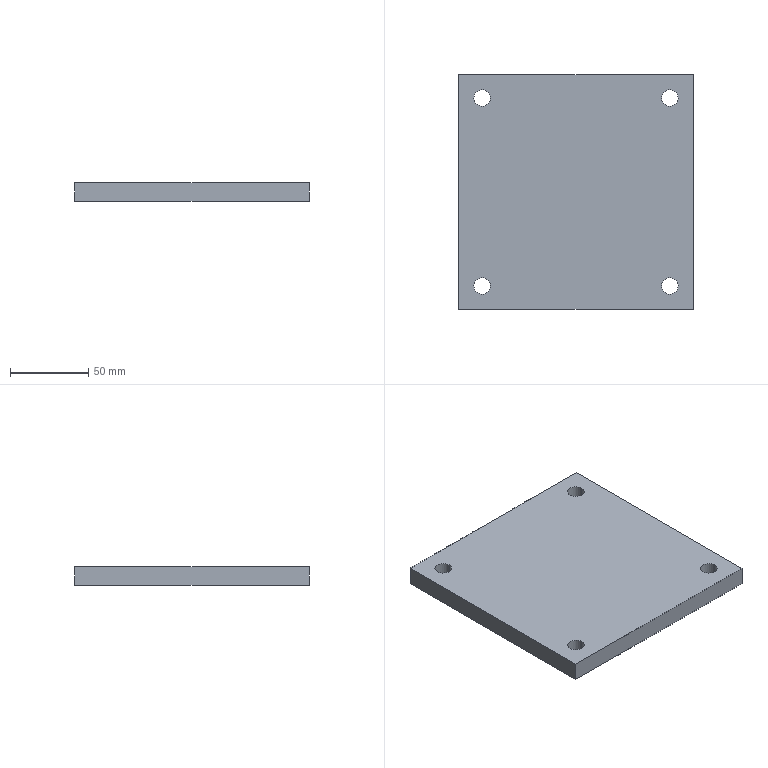Component | SolidWorks | CSFA2082 074-1 | 1 solid | 14 faces | box 150 x 150 x 12 mm | volume 265844 mm3 | cylinder 8 | plane 6 | commonest cylinder face diameters 10.5 x8
build123d program:
from build123d import *

# Parameters (mm, degrees)
SKETCH1_W                        = 150
SKETCH1_H                        = 150
EXTRUDE1_DEPTH                   = 12
F_10_5_10_5_DIAMETER_HOLE1_D     = 10.5
F_10_5_10_5_DIAMETER_HOLE1_DEPTH = 71
F_10_5_10_5_DIAMETER_HOLE1_TIP   = 3.155


with BuildPart() as part:
    # Sketch1 → Extrude1 (new body)
    with BuildSketch(Plane.XY):
        Rectangle(SKETCH1_W, SKETCH1_H)
    extrude(amount=EXTRUDE1_DEPTH)

    # 10.5 _10.5_ Diameter Hole1
    with Locations(Plane.XY.offset(12)):
        with Locations((-60, 60), (-60, -60), (60, -60), (60, 60)):
            Hole(F_10_5_10_5_DIAMETER_HOLE1_D / 2, depth=F_10_5_10_5_DIAMETER_HOLE1_DEPTH)
            with Locations((0, 0, -(F_10_5_10_5_DIAMETER_HOLE1_DEPTH + F_10_5_10_5_DIAMETER_HOLE1_TIP / 2))):  # 118° drill point
                Cone(0, F_10_5_10_5_DIAMETER_HOLE1_D / 2, F_10_5_10_5_DIAMETER_HOLE1_TIP, mode=Mode.SUBTRACT)


solid = part.part

# Placed as in the assembly
solid = solid.moved(Location((172.551, -218.176, 585), (0, 0, 0)))
STEP:
#1=COLOUR_RGB('',0.7922,0.8196,0.9333);
#2=FILL_AREA_STYLE_COLOUR('',#1);
#3=FILL_AREA_STYLE('',(#2));
#4=SURFACE_STYLE_FILL_AREA(#3);
#5=SURFACE_SIDE_STYLE('',(#4));
#6=SURFACE_STYLE_USAGE(.BOTH.,#5);
#7=PRESENTATION_STYLE_ASSIGNMENT((#6));
#8=CARTESIAN_POINT('',(4.638,-6.227,23.031));
#9=VERTEX_POINT('',#8);
#10=CARTESIAN_POINT('',(4.224,-6.227,23.031));
#11=VERTEX_POINT('',#10);
#12=CARTESIAN_POINT('',(4.431,-6.227,23.031));
#13=DIRECTION('',(0.,0.,-1.));
#14=DIRECTION('',(-1.,0.,0.));
#15=AXIS2_PLACEMENT_3D('',#12,#13,#14);
#16=CIRCLE('',#15,0.2067);
#17=EDGE_CURVE('',#9,#11,#16,.T.);
#18=ORIENTED_EDGE('',*,*,#17,.T.);
#19=CARTESIAN_POINT('',(4.224,-6.227,23.504));
#20=VERTEX_POINT('',#19);
#21=CARTESIAN_POINT('',(4.224,-6.227,23.504));
#22=DIRECTION('',(0.,0.,1.));
#23=VECTOR('',#22,39.37);
#24=LINE('',#21,#23);
#25=EDGE_CURVE('',#11,#20,#24,.T.);
#26=ORIENTED_EDGE('',*,*,#25,.T.);
#27=CARTESIAN_POINT('',(4.638,-6.227,23.504));
#28=VERTEX_POINT('',#27);
#29=CARTESIAN_POINT('',(4.431,-6.227,23.504));
#30=DIRECTION('',(0.,0.,1.));
#31=DIRECTION('',(1.,0.,0.));
#32=AXIS2_PLACEMENT_3D('',#29,#30,#31);
#33=CIRCLE('',#32,0.2067);
#34=EDGE_CURVE('',#20,#28,#33,.T.);
#35=ORIENTED_EDGE('',*,*,#34,.T.);
#36=CARTESIAN_POINT('',(4.638,-6.227,23.504));
#37=DIRECTION('',(0.,0.,1.));
#38=VECTOR('',#37,39.37);
#39=LINE('',#36,#38);
#40=EDGE_CURVE('',#9,#28,#39,.T.);
#41=ORIENTED_EDGE('',*,*,#40,.F.);
#42=EDGE_LOOP('',(#18,#26,#35,#41));
#43=FACE_OUTER_BOUND('',#42,.T.);
#44=CARTESIAN_POINT('',(4.431,-6.227,23.504));
#45=DIRECTION('',(0.,0.,1.));
#46=DIRECTION('',(1.,0.,0.));
#47=AXIS2_PLACEMENT_3D('',#44,#45,#46);
#48=CYLINDRICAL_SURFACE('',#47,0.2067);
#49=ADVANCED_FACE('',(#43),#48,.F.);
#50=CARTESIAN_POINT('',(4.638,-10.952,23.031));
#51=VERTEX_POINT('',#50);
#52=CARTESIAN_POINT('',(4.224,-10.952,23.031));
#53=VERTEX_POINT('',#52);
#54=CARTESIAN_POINT('',(4.431,-10.952,23.031));
#55=DIRECTION('',(0.,0.,-1.));
#56=DIRECTION('',(-1.,0.,0.));
#57=AXIS2_PLACEMENT_3D('',#54,#55,#56);
#58=CIRCLE('',#57,0.2067);
#59=EDGE_CURVE('',#51,#53,#58,.T.);
#60=ORIENTED_EDGE('',*,*,#59,.T.);
#61=CARTESIAN_POINT('',(4.224,-10.952,23.504));
#62=VERTEX_POINT('',#61);
#63=CARTESIAN_POINT('',(4.224,-10.952,23.504));
#64=DIRECTION('',(0.,0.,1.));
#65=VECTOR('',#64,39.37);
#66=LINE('',#63,#65);
#67=EDGE_CURVE('',#53,#62,#66,.T.);
#68=ORIENTED_EDGE('',*,*,#67,.T.);
#69=CARTESIAN_POINT('',(4.638,-10.952,23.504));
#70=VERTEX_POINT('',#69);
#71=CARTESIAN_POINT('',(4.431,-10.952,23.504));
#72=DIRECTION('',(0.,0.,1.));
#73=DIRECTION('',(1.,0.,0.));
#74=AXIS2_PLACEMENT_3D('',#71,#72,#73);
#75=CIRCLE('',#74,0.2067);
#76=EDGE_CURVE('',#62,#70,#75,.T.);
#77=ORIENTED_EDGE('',*,*,#76,.T.);
#78=CARTESIAN_POINT('',(4.638,-10.952,23.504));
#79=DIRECTION('',(0.,0.,1.));
#80=VECTOR('',#79,39.37);
#81=LINE('',#78,#80);
#82=EDGE_CURVE('',#51,#70,#81,.T.);
#83=ORIENTED_EDGE('',*,*,#82,.F.);
#84=EDGE_LOOP('',(#60,#68,#77,#83));
#85=FACE_OUTER_BOUND('',#84,.T.);
#86=CARTESIAN_POINT('',(4.431,-10.952,23.504));
#87=DIRECTION('',(0.,0.,1.));
#88=DIRECTION('',(1.,0.,0.));
#89=AXIS2_PLACEMENT_3D('',#86,#87,#88);
#90=CYLINDRICAL_SURFACE('',#89,0.2067);
#91=ADVANCED_FACE('',(#85),#90,.F.);
#92=CARTESIAN_POINT('',(9.362,-10.952,23.031));
#93=VERTEX_POINT('',#92);
#94=CARTESIAN_POINT('',(8.949,-10.952,23.031));
#95=VERTEX_POINT('',#94);
#96=CARTESIAN_POINT('',(9.156,-10.952,23.031));
#97=DIRECTION('',(0.,0.,-1.));
#98=DIRECTION('',(-1.,0.,0.));
#99=AXIS2_PLACEMENT_3D('',#96,#97,#98);
#100=CIRCLE('',#99,0.2067);
#101=EDGE_CURVE('',#93,#95,#100,.T.);
#102=ORIENTED_EDGE('',*,*,#101,.T.);
#103=CARTESIAN_POINT('',(8.949,-10.952,23.504));
#104=VERTEX_POINT('',#103);
#105=CARTESIAN_POINT('',(8.949,-10.952,23.504));
#106=DIRECTION('',(0.,0.,1.));
#107=VECTOR('',#106,39.37);
#108=LINE('',#105,#107);
#109=EDGE_CURVE('',#95,#104,#108,.T.);
#110=ORIENTED_EDGE('',*,*,#109,.T.);
#111=CARTESIAN_POINT('',(9.362,-10.952,23.504));
#112=VERTEX_POINT('',#111);
#113=CARTESIAN_POINT('',(9.156,-10.952,23.504));
#114=DIRECTION('',(0.,0.,1.));
#115=DIRECTION('',(1.,0.,0.));
#116=AXIS2_PLACEMENT_3D('',#113,#114,#115);
#117=CIRCLE('',#116,0.2067);
#118=EDGE_CURVE('',#104,#112,#117,.T.);
#119=ORIENTED_EDGE('',*,*,#118,.T.);
#120=CARTESIAN_POINT('',(9.362,-10.952,23.504));
#121=DIRECTION('',(0.,0.,1.));
#122=VECTOR('',#121,39.37);
#123=LINE('',#120,#122);
#124=EDGE_CURVE('',#93,#112,#123,.T.);
#125=ORIENTED_EDGE('',*,*,#124,.F.);
#126=EDGE_LOOP('',(#102,#110,#119,#125));
#127=FACE_OUTER_BOUND('',#126,.T.);
#128=CARTESIAN_POINT('',(9.156,-10.952,23.504));
#129=DIRECTION('',(0.,0.,1.));
#130=DIRECTION('',(1.,0.,0.));
#131=AXIS2_PLACEMENT_3D('',#128,#129,#130);
#132=CYLINDRICAL_SURFACE('',#131,0.2067);
#133=ADVANCED_FACE('',(#127),#132,.F.);
#134=CARTESIAN_POINT('',(9.362,-6.227,23.031));
#135=VERTEX_POINT('',#134);
#136=CARTESIAN_POINT('',(8.949,-6.227,23.031));
#137=VERTEX_POINT('',#136);
#138=CARTESIAN_POINT('',(9.156,-6.227,23.031));
#139=DIRECTION('',(0.,0.,-1.));
#140=DIRECTION('',(-1.,0.,0.));
#141=AXIS2_PLACEMENT_3D('',#138,#139,#140);
#142=CIRCLE('',#141,0.2067);
#143=EDGE_CURVE('',#135,#137,#142,.T.);
#144=ORIENTED_EDGE('',*,*,#143,.T.);
#145=CARTESIAN_POINT('',(8.949,-6.227,23.504));
#146=VERTEX_POINT('',#145);
#147=CARTESIAN_POINT('',(8.949,-6.227,23.504));
#148=DIRECTION('',(0.,0.,1.));
#149=VECTOR('',#148,39.37);
#150=LINE('',#147,#149);
#151=EDGE_CURVE('',#137,#146,#150,.T.);
#152=ORIENTED_EDGE('',*,*,#151,.T.);
#153=CARTESIAN_POINT('',(9.362,-6.227,23.504));
#154=VERTEX_POINT('',#153);
#155=CARTESIAN_POINT('',(9.156,-6.227,23.504));
#156=DIRECTION('',(0.,0.,1.));
#157=DIRECTION('',(1.,0.,0.));
#158=AXIS2_PLACEMENT_3D('',#155,#156,#157);
#159=CIRCLE('',#158,0.2067);
#160=EDGE_CURVE('',#146,#154,#159,.T.);
#161=ORIENTED_EDGE('',*,*,#160,.T.);
#162=CARTESIAN_POINT('',(9.362,-6.227,23.504));
#163=DIRECTION('',(0.,0.,1.));
#164=VECTOR('',#163,39.37);
#165=LINE('',#162,#164);
#166=EDGE_CURVE('',#135,#154,#165,.T.);
#167=ORIENTED_EDGE('',*,*,#166,.F.);
#168=EDGE_LOOP('',(#144,#152,#161,#167));
#169=FACE_OUTER_BOUND('',#168,.T.);
#170=CARTESIAN_POINT('',(9.156,-6.227,23.504));
#171=DIRECTION('',(0.,0.,1.));
#172=DIRECTION('',(1.,0.,0.));
#173=AXIS2_PLACEMENT_3D('',#170,#171,#172);
#174=CYLINDRICAL_SURFACE('',#173,0.2067);
#175=ADVANCED_FACE('',(#169),#174,.F.);
#176=CARTESIAN_POINT('',(9.746,-11.542,23.031));
#177=VERTEX_POINT('',#176);
#178=CARTESIAN_POINT('',(9.746,-5.637,23.031));
#179=VERTEX_POINT('',#178);
#180=CARTESIAN_POINT('',(9.746,-11.542,23.031));
#181=DIRECTION('',(0.,1.,0.));
#182=VECTOR('',#181,39.37);
#183=LINE('',#180,#182);
#184=EDGE_CURVE('',#177,#179,#183,.T.);
#185=ORIENTED_EDGE('',*,*,#184,.T.);
#186=CARTESIAN_POINT('',(9.746,-5.637,23.504));
#187=VERTEX_POINT('',#186);
#188=CARTESIAN_POINT('',(9.746,-5.637,23.504));
#189=DIRECTION('',(0.,0.,-1.));
#190=VECTOR('',#189,39.37);
#191=LINE('',#188,#190);
#192=EDGE_CURVE('',#187,#179,#191,.T.);
#193=ORIENTED_EDGE('',*,*,#192,.F.);
#194=CARTESIAN_POINT('',(9.746,-11.542,23.504));
#195=VERTEX_POINT('',#194);
#196=CARTESIAN_POINT('',(9.746,-11.542,23.504));
#197=DIRECTION('',(0.,1.,0.));
#198=VECTOR('',#197,39.37);
#199=LINE('',#196,#198);
#200=EDGE_CURVE('',#195,#187,#199,.T.);
#201=ORIENTED_EDGE('',*,*,#200,.F.);
#202=CARTESIAN_POINT('',(9.746,-11.542,23.504));
#203=DIRECTION('',(0.,0.,-1.));
#204=VECTOR('',#203,39.37);
#205=LINE('',#202,#204);
#206=EDGE_CURVE('',#195,#177,#205,.T.);
#207=ORIENTED_EDGE('',*,*,#206,.T.);
#208=EDGE_LOOP('',(#185,#193,#201,#207));
#209=FACE_OUTER_BOUND('',#208,.T.);
#210=CARTESIAN_POINT('',(9.746,-11.542,23.504));
#211=DIRECTION('',(-1.,0.,0.));
#212=DIRECTION('',(0.,0.,1.));
#213=AXIS2_PLACEMENT_3D('',#210,#211,#212);
#214=PLANE('',#213);
#215=ADVANCED_FACE('',(#209),#214,.F.);
#216=CARTESIAN_POINT('',(3.841,-5.637,23.031));
#217=VERTEX_POINT('',#216);
#218=CARTESIAN_POINT('',(3.841,-5.637,23.031));
#219=DIRECTION('',(-1.,0.,0.));
#220=VECTOR('',#219,39.37);
#221=LINE('',#218,#220);
#222=EDGE_CURVE('',#179,#217,#221,.T.);
#223=ORIENTED_EDGE('',*,*,#222,.T.);
#224=CARTESIAN_POINT('',(3.841,-5.637,23.504));
#225=VERTEX_POINT('',#224);
#226=CARTESIAN_POINT('',(3.841,-5.637,23.504));
#227=DIRECTION('',(0.,0.,-1.));
#228=VECTOR('',#227,39.37);
#229=LINE('',#226,#228);
#230=EDGE_CURVE('',#225,#217,#229,.T.);
#231=ORIENTED_EDGE('',*,*,#230,.F.);
#232=CARTESIAN_POINT('',(3.841,-5.637,23.504));
#233=DIRECTION('',(-1.,0.,0.));
#234=VECTOR('',#233,39.37);
#235=LINE('',#232,#234);
#236=EDGE_CURVE('',#187,#225,#235,.T.);
#237=ORIENTED_EDGE('',*,*,#236,.F.);
#238=ORIENTED_EDGE('',*,*,#192,.T.);
#239=EDGE_LOOP('',(#223,#231,#237,#238));
#240=FACE_OUTER_BOUND('',#239,.T.);
#241=CARTESIAN_POINT('',(3.841,-5.637,23.504));
#242=DIRECTION('',(0.,-1.,0.));
#243=DIRECTION('',(0.,0.,-1.));
#244=AXIS2_PLACEMENT_3D('',#241,#242,#243);
#245=PLANE('',#244);
#246=ADVANCED_FACE('',(#240),#245,.F.);
#247=CARTESIAN_POINT('',(3.841,-11.542,23.031));
#248=VERTEX_POINT('',#247);
#249=CARTESIAN_POINT('',(3.841,-11.542,23.031));
#250=DIRECTION('',(0.,-1.,0.));
#251=VECTOR('',#250,39.37);
#252=LINE('',#249,#251);
#253=EDGE_CURVE('',#217,#248,#252,.T.);
#254=ORIENTED_EDGE('',*,*,#253,.T.);
#255=CARTESIAN_POINT('',(3.841,-11.542,23.504));
#256=VERTEX_POINT('',#255);
#257=CARTESIAN_POINT('',(3.841,-11.542,23.504));
#258=DIRECTION('',(0.,0.,-1.));
#259=VECTOR('',#258,39.37);
#260=LINE('',#257,#259);
#261=EDGE_CURVE('',#256,#248,#260,.T.);
#262=ORIENTED_EDGE('',*,*,#261,.F.);
#263=CARTESIAN_POINT('',(3.841,-11.542,23.504));
#264=DIRECTION('',(0.,-1.,0.));
#265=VECTOR('',#264,39.37);
#266=LINE('',#263,#265);
#267=EDGE_CURVE('',#225,#256,#266,.T.);
#268=ORIENTED_EDGE('',*,*,#267,.F.);
#269=ORIENTED_EDGE('',*,*,#230,.T.);
#270=EDGE_LOOP('',(#254,#262,#268,#269));
#271=FACE_OUTER_BOUND('',#270,.T.);
#272=CARTESIAN_POINT('',(3.841,-11.542,23.504));
#273=DIRECTION('',(1.,0.,0.));
#274=DIRECTION('',(0.,0.,-1.));
#275=AXIS2_PLACEMENT_3D('',#272,#273,#274);
#276=PLANE('',#275);
#277=ADVANCED_FACE('',(#271),#276,.F.);
#278=CARTESIAN_POINT('',(3.841,-11.542,23.031));
#279=DIRECTION('',(1.,0.,0.));
#280=VECTOR('',#279,39.37);
#281=LINE('',#278,#280);
#282=EDGE_CURVE('',#248,#177,#281,.T.);
#283=ORIENTED_EDGE('',*,*,#282,.T.);
#284=ORIENTED_EDGE('',*,*,#206,.F.);
#285=CARTESIAN_POINT('',(3.841,-11.542,23.504));
#286=DIRECTION('',(1.,0.,0.));
#287=VECTOR('',#286,39.37);
#288=LINE('',#285,#287);
#289=EDGE_CURVE('',#256,#195,#288,.T.);
#290=ORIENTED_EDGE('',*,*,#289,.F.);
#291=ORIENTED_EDGE('',*,*,#261,.T.);
#292=EDGE_LOOP('',(#283,#284,#290,#291));
#293=FACE_OUTER_BOUND('',#292,.T.);
#294=CARTESIAN_POINT('',(3.841,-11.542,23.504));
#295=DIRECTION('',(0.,1.,0.));
#296=DIRECTION('',(0.,0.,1.));
#297=AXIS2_PLACEMENT_3D('',#294,#295,#296);
#298=PLANE('',#297);
#299=ADVANCED_FACE('',(#293),#298,.F.);
#300=CARTESIAN_POINT('',(4.431,-6.227,23.504));
#301=DIRECTION('',(0.,0.,1.));
#302=DIRECTION('',(1.,0.,0.));
#303=AXIS2_PLACEMENT_3D('',#300,#301,#302);
#304=CIRCLE('',#303,0.2067);
#305=EDGE_CURVE('',#28,#20,#304,.T.);
#306=ORIENTED_EDGE('',*,*,#305,.F.);
#307=ORIENTED_EDGE('',*,*,#34,.F.);
#308=EDGE_LOOP('',(#306,#307));
#309=FACE_BOUND('',#308,.T.);
#310=CARTESIAN_POINT('',(4.431,-10.952,23.504));
#311=DIRECTION('',(0.,0.,1.));
#312=DIRECTION('',(1.,0.,0.));
#313=AXIS2_PLACEMENT_3D('',#310,#311,#312);
#314=CIRCLE('',#313,0.2067);
#315=EDGE_CURVE('',#70,#62,#314,.T.);
#316=ORIENTED_EDGE('',*,*,#315,.F.);
#317=ORIENTED_EDGE('',*,*,#76,.F.);
#318=EDGE_LOOP('',(#316,#317));
#319=FACE_BOUND('',#318,.T.);
#320=CARTESIAN_POINT('',(9.156,-10.952,23.504));
#321=DIRECTION('',(0.,0.,1.));
#322=DIRECTION('',(1.,0.,0.));
#323=AXIS2_PLACEMENT_3D('',#320,#321,#322);
#324=CIRCLE('',#323,0.2067);
#325=EDGE_CURVE('',#112,#104,#324,.T.);
#326=ORIENTED_EDGE('',*,*,#325,.F.);
#327=ORIENTED_EDGE('',*,*,#118,.F.);
#328=EDGE_LOOP('',(#326,#327));
#329=FACE_BOUND('',#328,.T.);
#330=CARTESIAN_POINT('',(9.156,-6.227,23.504));
#331=DIRECTION('',(0.,0.,1.));
#332=DIRECTION('',(1.,0.,0.));
#333=AXIS2_PLACEMENT_3D('',#330,#331,#332);
#334=CIRCLE('',#333,0.2067);
#335=EDGE_CURVE('',#154,#146,#334,.T.);
#336=ORIENTED_EDGE('',*,*,#335,.F.);
#337=ORIENTED_EDGE('',*,*,#160,.F.);
#338=EDGE_LOOP('',(#336,#337));
#339=FACE_BOUND('',#338,.T.);
#340=ORIENTED_EDGE('',*,*,#200,.T.);
#341=ORIENTED_EDGE('',*,*,#236,.T.);
#342=ORIENTED_EDGE('',*,*,#267,.T.);
#343=ORIENTED_EDGE('',*,*,#289,.T.);
#344=EDGE_LOOP('',(#340,#341,#342,#343));
#345=FACE_OUTER_BOUND('',#344,.T.);
#346=CARTESIAN_POINT('',(9.746,-5.637,23.504));
#347=DIRECTION('',(0.,0.,-1.));
#348=DIRECTION('',(-1.,0.,0.));
#349=AXIS2_PLACEMENT_3D('',#346,#347,#348);
#350=PLANE('',#349);
#351=ADVANCED_FACE('',(#309,#319,#329,#339,#345),#350,.F.);
#352=ORIENTED_EDGE('',*,*,#17,.F.);
#353=CARTESIAN_POINT('',(4.431,-6.227,23.031));
#354=DIRECTION('',(0.,0.,-1.));
#355=DIRECTION('',(-1.,0.,0.));
#356=AXIS2_PLACEMENT_3D('',#353,#354,#355);
#357=CIRCLE('',#356,0.2067);
#358=EDGE_CURVE('',#11,#9,#357,.T.);
#359=ORIENTED_EDGE('',*,*,#358,.F.);
#360=EDGE_LOOP('',(#352,#359));
#361=FACE_BOUND('',#360,.T.);
#362=ORIENTED_EDGE('',*,*,#59,.F.);
#363=CARTESIAN_POINT('',(4.431,-10.952,23.031));
#364=DIRECTION('',(0.,0.,-1.));
#365=DIRECTION('',(-1.,0.,0.));
#366=AXIS2_PLACEMENT_3D('',#363,#364,#365);
#367=CIRCLE('',#366,0.2067);
#368=EDGE_CURVE('',#53,#51,#367,.T.);
#369=ORIENTED_EDGE('',*,*,#368,.F.);
#370=EDGE_LOOP('',(#362,#369));
#371=FACE_BOUND('',#370,.T.);
#372=ORIENTED_EDGE('',*,*,#101,.F.);
#373=CARTESIAN_POINT('',(9.156,-10.952,23.031));
#374=DIRECTION('',(0.,0.,-1.));
#375=DIRECTION('',(-1.,0.,0.));
#376=AXIS2_PLACEMENT_3D('',#373,#374,#375);
#377=CIRCLE('',#376,0.2067);
#378=EDGE_CURVE('',#95,#93,#377,.T.);
#379=ORIENTED_EDGE('',*,*,#378,.F.);
#380=EDGE_LOOP('',(#372,#379));
#381=FACE_BOUND('',#380,.T.);
#382=ORIENTED_EDGE('',*,*,#143,.F.);
#383=CARTESIAN_POINT('',(9.156,-6.227,23.031));
#384=DIRECTION('',(0.,0.,-1.));
#385=DIRECTION('',(-1.,0.,0.));
#386=AXIS2_PLACEMENT_3D('',#383,#384,#385);
#387=CIRCLE('',#386,0.2067);
#388=EDGE_CURVE('',#137,#135,#387,.T.);
#389=ORIENTED_EDGE('',*,*,#388,.F.);
#390=EDGE_LOOP('',(#382,#389));
#391=FACE_BOUND('',#390,.T.);
#392=ORIENTED_EDGE('',*,*,#184,.F.);
#393=ORIENTED_EDGE('',*,*,#282,.F.);
#394=ORIENTED_EDGE('',*,*,#253,.F.);
#395=ORIENTED_EDGE('',*,*,#222,.F.);
#396=EDGE_LOOP('',(#392,#393,#394,#395));
#397=FACE_OUTER_BOUND('',#396,.T.);
#398=CARTESIAN_POINT('',(9.746,-5.637,23.031));
#399=DIRECTION('',(0.,0.,-1.));
#400=DIRECTION('',(-1.,0.,0.));
#401=AXIS2_PLACEMENT_3D('',#398,#399,#400);
#402=PLANE('',#401);
#403=ADVANCED_FACE('',(#361,#371,#381,#391,#397),#402,.T.);
#404=ORIENTED_EDGE('',*,*,#151,.F.);
#405=ORIENTED_EDGE('',*,*,#388,.T.);
#406=ORIENTED_EDGE('',*,*,#166,.T.);
#407=ORIENTED_EDGE('',*,*,#335,.T.);
#408=EDGE_LOOP('',(#404,#405,#406,#407));
#409=FACE_OUTER_BOUND('',#408,.T.);
#410=CARTESIAN_POINT('',(9.156,-6.227,23.504));
#411=DIRECTION('',(0.,0.,1.));
#412=DIRECTION('',(1.,0.,0.));
#413=AXIS2_PLACEMENT_3D('',#410,#411,#412);
#414=CYLINDRICAL_SURFACE('',#413,0.2067);
#415=ADVANCED_FACE('',(#409),#414,.F.);
#416=ORIENTED_EDGE('',*,*,#109,.F.);
#417=ORIENTED_EDGE('',*,*,#378,.T.);
#418=ORIENTED_EDGE('',*,*,#124,.T.);
#419=ORIENTED_EDGE('',*,*,#325,.T.);
#420=EDGE_LOOP('',(#416,#417,#418,#419));
#421=FACE_OUTER_BOUND('',#420,.T.);
#422=CARTESIAN_POINT('',(9.156,-10.952,23.504));
#423=DIRECTION('',(0.,0.,1.));
#424=DIRECTION('',(1.,0.,0.));
#425=AXIS2_PLACEMENT_3D('',#422,#423,#424);
#426=CYLINDRICAL_SURFACE('',#425,0.2067);
#427=ADVANCED_FACE('',(#421),#426,.F.);
#428=ORIENTED_EDGE('',*,*,#67,.F.);
#429=ORIENTED_EDGE('',*,*,#368,.T.);
#430=ORIENTED_EDGE('',*,*,#82,.T.);
#431=ORIENTED_EDGE('',*,*,#315,.T.);
#432=EDGE_LOOP('',(#428,#429,#430,#431));
#433=FACE_OUTER_BOUND('',#432,.T.);
#434=CARTESIAN_POINT('',(4.431,-10.952,23.504));
#435=DIRECTION('',(0.,0.,1.));
#436=DIRECTION('',(1.,0.,0.));
#437=AXIS2_PLACEMENT_3D('',#434,#435,#436);
#438=CYLINDRICAL_SURFACE('',#437,0.2067);
#439=ADVANCED_FACE('',(#433),#438,.F.);
#440=ORIENTED_EDGE('',*,*,#25,.F.);
#441=ORIENTED_EDGE('',*,*,#358,.T.);
#442=ORIENTED_EDGE('',*,*,#40,.T.);
#443=ORIENTED_EDGE('',*,*,#305,.T.);
#444=EDGE_LOOP('',(#440,#441,#442,#443));
#445=FACE_OUTER_BOUND('',#444,.T.);
#446=CARTESIAN_POINT('',(4.431,-6.227,23.504));
#447=DIRECTION('',(0.,0.,1.));
#448=DIRECTION('',(1.,0.,0.));
#449=AXIS2_PLACEMENT_3D('',#446,#447,#448);
#450=CYLINDRICAL_SURFACE('',#449,0.2067);
#451=ADVANCED_FACE('',(#445),#450,.F.);
#452=CLOSED_SHELL('',(#49,#91,#133,#175,#215,#246,#277,#299,#351,#403,#415,#427,#439,#451));
#453=MANIFOLD_SOLID_BREP('',#452);
#454=STYLED_ITEM('',(#7),#453);
#455=(LENGTH_UNIT()NAMED_UNIT(*)SI_UNIT($,.METRE.));
#456=LENGTH_MEASURE_WITH_UNIT(LENGTH_MEASURE(0.0254),#455);
#457=DIMENSIONAL_EXPONENTS(1.,0.,0.,0.,0.,0.,0.);
#458=(CONVERSION_BASED_UNIT('',#456)LENGTH_UNIT()NAMED_UNIT(#457));
#459=UNCERTAINTY_MEASURE_WITH_UNIT(LENGTH_MEASURE(0.00001),#458,'','');
#460=(NAMED_UNIT(*)PLANE_ANGLE_UNIT()SI_UNIT($,.RADIAN.));
#461=(NAMED_UNIT(*)SI_UNIT($,.STERADIAN.)SOLID_ANGLE_UNIT());
#462=(GEOMETRIC_REPRESENTATION_CONTEXT(3)GLOBAL_UNCERTAINTY_ASSIGNED_CONTEXT((#459))GLOBAL_UNIT_ASSIGNED_CONTEXT((#458,#460,#461))REPRESENTATION_CONTEXT('',''));
#463=MECHANICAL_DESIGN_GEOMETRIC_PRESENTATION_REPRESENTATION('',(#454),#462);
#464=PRESENTATION_LAYER_ASSIGNMENT('','',(#454));
#465=CARTESIAN_POINT('',(0.,0.,0.));
#466=DIRECTION('',(0.,0.,1.));
#467=DIRECTION('',(1.,0.,0.));
#468=AXIS2_PLACEMENT_3D('',#465,#466,#467);
#469=(LENGTH_UNIT()NAMED_UNIT(*)SI_UNIT($,.METRE.));
#470=LENGTH_MEASURE_WITH_UNIT(LENGTH_MEASURE(0.0254),#469);
#471=DIMENSIONAL_EXPONENTS(1.,0.,0.,0.,0.,0.,0.);
#472=(CONVERSION_BASED_UNIT('',#470)LENGTH_UNIT()NAMED_UNIT(#471));
#473=UNCERTAINTY_MEASURE_WITH_UNIT(LENGTH_MEASURE(0.00001),#472,'','');
#474=(NAMED_UNIT(*)PLANE_ANGLE_UNIT()SI_UNIT($,.RADIAN.));
#475=(NAMED_UNIT(*)SI_UNIT($,.STERADIAN.)SOLID_ANGLE_UNIT());
#476=(GEOMETRIC_REPRESENTATION_CONTEXT(3)GLOBAL_UNCERTAINTY_ASSIGNED_CONTEXT((#473))GLOBAL_UNIT_ASSIGNED_CONTEXT((#472,#474,#475))REPRESENTATION_CONTEXT('',''));
#477=ADVANCED_BREP_SHAPE_REPRESENTATION('',(#453,#468),#476);